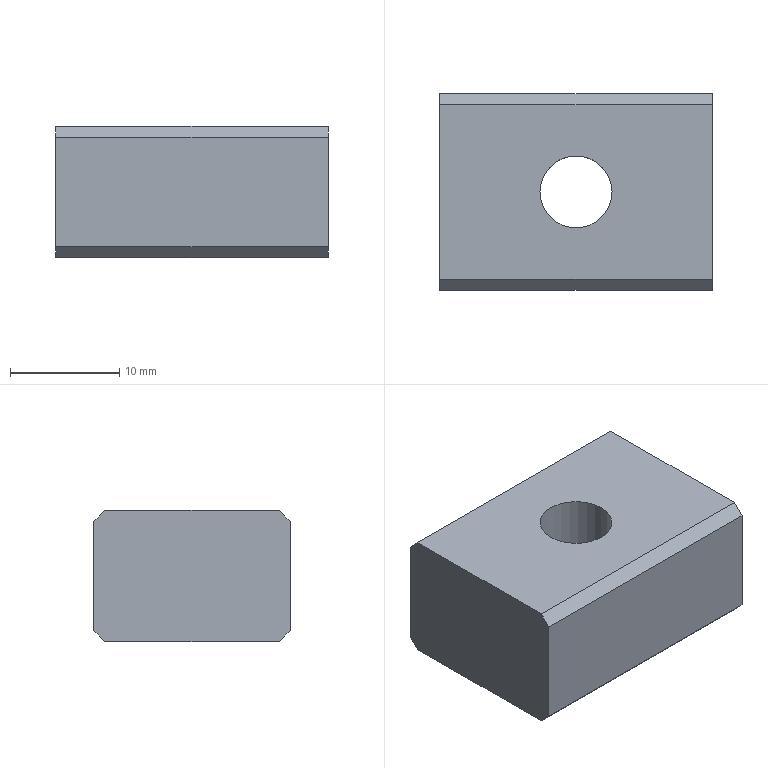Component | NX | LOCATING_KEY | 1 solid | 13 faces | box 25 x 18 x 12 mm | volume 4526 mm3 | plane 11 | cylinder 2 | commonest cylinder face diameters 6.6 x1 11 x1
STEP:
#1=CARTESIAN_POINT('',(0.,0.,0.));
#2=DIRECTION('',(0.,0.,1.));
#3=DIRECTION('',(1.,0.,0.));
#4=AXIS2_PLACEMENT_3D('',#1,#2,#3);
#5=CARTESIAN_POINT('',(195.,99.,29.));
#6=VERTEX_POINT('',#5);
#7=CARTESIAN_POINT('',(195.,99.,19.));
#8=VERTEX_POINT('',#7);
#9=CARTESIAN_POINT('',(195.,99.,30.));
#10=DIRECTION('',(0.,0.,-1.));
#11=VECTOR('',#10,1.);
#12=LINE('',#9,#11);
#13=CARTESIAN_POINT('',(195.,99.,30.));
#14=DIRECTION('',(1.,0.,0.));
#15=DIRECTION('',(0.,0.,-1.));
#16=AXIS2_PLACEMENT_3D('',#13,#14,#15);
#17=PLANE('',#16);
#18=CARTESIAN_POINT('',(0.,0.));
#19=DIRECTION('',(1.,0.));
#20=VECTOR('',#19,1.);
#21=LINE('',#18,#20);
#22=(GEOMETRIC_REPRESENTATION_CONTEXT(2)PARAMETRIC_REPRESENTATION_CONTEXT()REPRESENTATION_CONTEXT('',''));
#23=DEFINITIONAL_REPRESENTATION('',(#21),#22);
#24=PCURVE('',#17,#23);
#25=CARTESIAN_POINT('',(220.,99.,30.));
#26=DIRECTION('',(0.,-1.,0.));
#27=DIRECTION('',(0.,0.,-1.));
#28=AXIS2_PLACEMENT_3D('',#25,#26,#27);
#29=PLANE('',#28);
#30=CARTESIAN_POINT('',(0.,-25.));
#31=DIRECTION('',(1.,0.));
#32=VECTOR('',#31,1.);
#33=LINE('',#30,#32);
#34=(GEOMETRIC_REPRESENTATION_CONTEXT(2)PARAMETRIC_REPRESENTATION_CONTEXT()REPRESENTATION_CONTEXT('',''));
#35=DEFINITIONAL_REPRESENTATION('',(#33),#34);
#36=PCURVE('',#29,#35);
#37=SURFACE_CURVE('',#12,(#24,#36),.PCURVE_S1.);
#38=EDGE_CURVE('',#6,#8,#37,.T.);
#39=ORIENTED_EDGE('',*,*,#38,.T.);
#40=CARTESIAN_POINT('',(195.,98.,18.));
#41=VERTEX_POINT('',#40);
#42=CARTESIAN_POINT('',(195.,99.,19.));
#43=DIRECTION('',(0.,-0.7071,-0.7071));
#44=VECTOR('',#43,1.);
#45=LINE('',#42,#44);
#46=CARTESIAN_POINT('',(11.,0.));
#47=DIRECTION('',(0.7071,-0.7071));
#48=VECTOR('',#47,1.);
#49=LINE('',#46,#48);
#50=(GEOMETRIC_REPRESENTATION_CONTEXT(2)PARAMETRIC_REPRESENTATION_CONTEXT()REPRESENTATION_CONTEXT('',''));
#51=DEFINITIONAL_REPRESENTATION('',(#49),#50);
#52=PCURVE('',#17,#51);
#53=CARTESIAN_POINT('',(220.,99.,19.));
#54=DIRECTION('',(0.,-0.7071,0.7071));
#55=DIRECTION('',(-1.,0.,0.));
#56=AXIS2_PLACEMENT_3D('',#53,#54,#55);
#57=PLANE('',#56);
#58=CARTESIAN_POINT('',(25.,0.));
#59=DIRECTION('',(0.,1.));
#60=VECTOR('',#59,1.);
#61=LINE('',#58,#60);
#62=(GEOMETRIC_REPRESENTATION_CONTEXT(2)PARAMETRIC_REPRESENTATION_CONTEXT()REPRESENTATION_CONTEXT('',''));
#63=DEFINITIONAL_REPRESENTATION('',(#61),#62);
#64=PCURVE('',#57,#63);
#65=SURFACE_CURVE('',#45,(#52,#64),.PCURVE_S1.);
#66=EDGE_CURVE('',#8,#41,#65,.T.);
#67=ORIENTED_EDGE('',*,*,#66,.T.);
#68=CARTESIAN_POINT('',(195.,82.,18.));
#69=VERTEX_POINT('',#68);
#70=CARTESIAN_POINT('',(195.,99.,18.));
#71=DIRECTION('',(0.,-1.,0.));
#72=VECTOR('',#71,1.);
#73=LINE('',#70,#72);
#74=CARTESIAN_POINT('',(12.,0.));
#75=DIRECTION('',(0.,-1.));
#76=VECTOR('',#75,1.);
#77=LINE('',#74,#76);
#78=(GEOMETRIC_REPRESENTATION_CONTEXT(2)PARAMETRIC_REPRESENTATION_CONTEXT()REPRESENTATION_CONTEXT('',''));
#79=DEFINITIONAL_REPRESENTATION('',(#77),#78);
#80=PCURVE('',#17,#79);
#81=CARTESIAN_POINT('',(207.5,90.,18.));
#82=DIRECTION('',(0.,0.,1.));
#83=DIRECTION('',(1.,0.,0.));
#84=AXIS2_PLACEMENT_3D('',#81,#82,#83);
#85=PLANE('',#84);
#86=CARTESIAN_POINT('',(-12.5,9.));
#87=DIRECTION('',(0.,-1.));
#88=VECTOR('',#87,1.);
#89=LINE('',#86,#88);
#90=(GEOMETRIC_REPRESENTATION_CONTEXT(2)PARAMETRIC_REPRESENTATION_CONTEXT()REPRESENTATION_CONTEXT('',''));
#91=DEFINITIONAL_REPRESENTATION('',(#89),#90);
#92=PCURVE('',#85,#91);
#93=SURFACE_CURVE('',#73,(#80,#92),.PCURVE_S1.);
#94=EDGE_CURVE('',#41,#69,#93,.T.);
#95=ORIENTED_EDGE('',*,*,#94,.T.);
#96=CARTESIAN_POINT('',(195.,81.,19.));
#97=VERTEX_POINT('',#96);
#98=CARTESIAN_POINT('',(195.,81.,19.));
#99=DIRECTION('',(0.,-0.7071,0.7071));
#100=VECTOR('',#99,1.);
#101=LINE('',#98,#100);
#102=CARTESIAN_POINT('',(11.,-18.));
#103=DIRECTION('',(-0.7071,-0.7071));
#104=VECTOR('',#103,1.);
#105=LINE('',#102,#104);
#106=(GEOMETRIC_REPRESENTATION_CONTEXT(2)PARAMETRIC_REPRESENTATION_CONTEXT()REPRESENTATION_CONTEXT('',''));
#107=DEFINITIONAL_REPRESENTATION('',(#105),#106);
#108=PCURVE('',#17,#107);
#109=CARTESIAN_POINT('',(195.,81.,19.));
#110=DIRECTION('',(0.,0.7071,0.7071));
#111=DIRECTION('',(1.,0.,0.));
#112=AXIS2_PLACEMENT_3D('',#109,#110,#111);
#113=PLANE('',#112);
#114=CARTESIAN_POINT('',(0.,0.));
#115=DIRECTION('',(0.,-1.));
#116=VECTOR('',#115,1.);
#117=LINE('',#114,#116);
#118=(GEOMETRIC_REPRESENTATION_CONTEXT(2)PARAMETRIC_REPRESENTATION_CONTEXT()REPRESENTATION_CONTEXT('',''));
#119=DEFINITIONAL_REPRESENTATION('',(#117),#118);
#120=PCURVE('',#113,#119);
#121=SURFACE_CURVE('',#101,(#108,#120),.PCURVE_S1.);
#122=EDGE_CURVE('',#69,#97,#121,.T.);
#123=ORIENTED_EDGE('',*,*,#122,.T.);
#124=CARTESIAN_POINT('',(195.,81.,29.));
#125=VERTEX_POINT('',#124);
#126=CARTESIAN_POINT('',(195.,81.,30.));
#127=DIRECTION('',(0.,0.,-1.));
#128=VECTOR('',#127,1.);
#129=LINE('',#126,#128);
#130=CARTESIAN_POINT('',(0.,-18.));
#131=DIRECTION('',(1.,0.));
#132=VECTOR('',#131,1.);
#133=LINE('',#130,#132);
#134=(GEOMETRIC_REPRESENTATION_CONTEXT(2)PARAMETRIC_REPRESENTATION_CONTEXT()REPRESENTATION_CONTEXT('',''));
#135=DEFINITIONAL_REPRESENTATION('',(#133),#134);
#136=PCURVE('',#17,#135);
#137=CARTESIAN_POINT('',(195.,81.,30.));
#138=DIRECTION('',(0.,1.,0.));
#139=DIRECTION('',(0.,0.,1.));
#140=AXIS2_PLACEMENT_3D('',#137,#138,#139);
#141=PLANE('',#140);
#142=CARTESIAN_POINT('',(0.,0.));
#143=DIRECTION('',(-1.,0.));
#144=VECTOR('',#143,1.);
#145=LINE('',#142,#144);
#146=(GEOMETRIC_REPRESENTATION_CONTEXT(2)PARAMETRIC_REPRESENTATION_CONTEXT()REPRESENTATION_CONTEXT('',''));
#147=DEFINITIONAL_REPRESENTATION('',(#145),#146);
#148=PCURVE('',#141,#147);
#149=SURFACE_CURVE('',#129,(#136,#148),.PCURVE_S1.);
#150=EDGE_CURVE('',#125,#97,#149,.T.);
#151=ORIENTED_EDGE('',*,*,#150,.F.);
#152=CARTESIAN_POINT('',(195.,82.,30.));
#153=VERTEX_POINT('',#152);
#154=CARTESIAN_POINT('',(195.,82.,30.));
#155=DIRECTION('',(0.,0.7071,0.7071));
#156=VECTOR('',#155,1.);
#157=LINE('',#154,#156);
#158=CARTESIAN_POINT('',(0.,-17.));
#159=DIRECTION('',(-0.7071,0.7071));
#160=VECTOR('',#159,1.);
#161=LINE('',#158,#160);
#162=(GEOMETRIC_REPRESENTATION_CONTEXT(2)PARAMETRIC_REPRESENTATION_CONTEXT()REPRESENTATION_CONTEXT('',''));
#163=DEFINITIONAL_REPRESENTATION('',(#161),#162);
#164=PCURVE('',#17,#163);
#165=CARTESIAN_POINT('',(207.5,82.,30.));
#166=DIRECTION('',(0.,-0.7071,0.7071));
#167=DIRECTION('',(-1.,0.,0.));
#168=AXIS2_PLACEMENT_3D('',#165,#166,#167);
#169=PLANE('',#168);
#170=CARTESIAN_POINT('',(12.5,0.));
#171=DIRECTION('',(0.,-1.));
#172=VECTOR('',#171,1.);
#173=LINE('',#170,#172);
#174=(GEOMETRIC_REPRESENTATION_CONTEXT(2)PARAMETRIC_REPRESENTATION_CONTEXT()REPRESENTATION_CONTEXT('',''));
#175=DEFINITIONAL_REPRESENTATION('',(#173),#174);
#176=PCURVE('',#169,#175);
#177=SURFACE_CURVE('',#157,(#164,#176),.PCURVE_S1.);
#178=EDGE_CURVE('',#125,#153,#177,.T.);
#179=ORIENTED_EDGE('',*,*,#178,.T.);
#180=CARTESIAN_POINT('',(195.,98.,30.));
#181=VERTEX_POINT('',#180);
#182=CARTESIAN_POINT('',(195.,99.,30.));
#183=DIRECTION('',(0.,-1.,0.));
#184=VECTOR('',#183,1.);
#185=LINE('',#182,#184);
#186=CARTESIAN_POINT('',(0.,0.));
#187=DIRECTION('',(0.,-1.));
#188=VECTOR('',#187,1.);
#189=LINE('',#186,#188);
#190=(GEOMETRIC_REPRESENTATION_CONTEXT(2)PARAMETRIC_REPRESENTATION_CONTEXT()REPRESENTATION_CONTEXT('',''));
#191=DEFINITIONAL_REPRESENTATION('',(#189),#190);
#192=PCURVE('',#17,#191);
#193=CARTESIAN_POINT('',(207.5,90.,30.));
#194=DIRECTION('',(0.,0.,1.));
#195=DIRECTION('',(1.,0.,0.));
#196=AXIS2_PLACEMENT_3D('',#193,#194,#195);
#197=PLANE('',#196);
#198=CARTESIAN_POINT('',(-12.5,9.));
#199=DIRECTION('',(0.,-1.));
#200=VECTOR('',#199,1.);
#201=LINE('',#198,#200);
#202=(GEOMETRIC_REPRESENTATION_CONTEXT(2)PARAMETRIC_REPRESENTATION_CONTEXT()REPRESENTATION_CONTEXT('',''));
#203=DEFINITIONAL_REPRESENTATION('',(#201),#202);
#204=PCURVE('',#197,#203);
#205=SURFACE_CURVE('',#185,(#192,#204),.PCURVE_S1.);
#206=EDGE_CURVE('',#181,#153,#205,.T.);
#207=ORIENTED_EDGE('',*,*,#206,.F.);
#208=CARTESIAN_POINT('',(195.,98.,30.));
#209=DIRECTION('',(0.,0.7071,-0.7071));
#210=VECTOR('',#209,1.);
#211=LINE('',#208,#210);
#212=CARTESIAN_POINT('',(0.,-1.));
#213=DIRECTION('',(0.7071,0.7071));
#214=VECTOR('',#213,1.);
#215=LINE('',#212,#214);
#216=(GEOMETRIC_REPRESENTATION_CONTEXT(2)PARAMETRIC_REPRESENTATION_CONTEXT()REPRESENTATION_CONTEXT('',''));
#217=DEFINITIONAL_REPRESENTATION('',(#215),#216);
#218=PCURVE('',#17,#217);
#219=CARTESIAN_POINT('',(207.5,98.,30.));
#220=DIRECTION('',(0.,0.7071,0.7071));
#221=DIRECTION('',(1.,0.,0.));
#222=AXIS2_PLACEMENT_3D('',#219,#220,#221);
#223=PLANE('',#222);
#224=CARTESIAN_POINT('',(-12.5,0.));
#225=DIRECTION('',(0.,1.));
#226=VECTOR('',#225,1.);
#227=LINE('',#224,#226);
#228=(GEOMETRIC_REPRESENTATION_CONTEXT(2)PARAMETRIC_REPRESENTATION_CONTEXT()REPRESENTATION_CONTEXT('',''));
#229=DEFINITIONAL_REPRESENTATION('',(#227),#228);
#230=PCURVE('',#223,#229);
#231=SURFACE_CURVE('',#211,(#218,#230),.PCURVE_S1.);
#232=EDGE_CURVE('',#181,#6,#231,.T.);
#233=ORIENTED_EDGE('',*,*,#232,.T.);
#234=EDGE_LOOP('',(#39,#67,#95,#123,#151,#179,#207,#233));
#235=FACE_BOUND('',#234,.T.);
#236=ADVANCED_FACE('',(#235),#17,.F.);
#237=ORIENTED_EDGE('',*,*,#150,.T.);
#238=CARTESIAN_POINT('',(220.,81.,19.));
#239=VERTEX_POINT('',#238);
#240=CARTESIAN_POINT('',(195.,81.,19.));
#241=DIRECTION('',(1.,0.,0.));
#242=VECTOR('',#241,1.);
#243=LINE('',#240,#242);
#244=CARTESIAN_POINT('',(-11.,0.));
#245=DIRECTION('',(0.,1.));
#246=VECTOR('',#245,1.);
#247=LINE('',#244,#246);
#248=(GEOMETRIC_REPRESENTATION_CONTEXT(2)PARAMETRIC_REPRESENTATION_CONTEXT()REPRESENTATION_CONTEXT('',''));
#249=DEFINITIONAL_REPRESENTATION('',(#247),#248);
#250=PCURVE('',#141,#249);
#251=CARTESIAN_POINT('',(0.,0.));
#252=DIRECTION('',(1.,0.));
#253=VECTOR('',#252,1.);
#254=LINE('',#251,#253);
#255=(GEOMETRIC_REPRESENTATION_CONTEXT(2)PARAMETRIC_REPRESENTATION_CONTEXT()REPRESENTATION_CONTEXT('',''));
#256=DEFINITIONAL_REPRESENTATION('',(#254),#255);
#257=PCURVE('',#113,#256);
#258=SURFACE_CURVE('',#243,(#250,#257),.PCURVE_S1.);
#259=EDGE_CURVE('',#97,#239,#258,.T.);
#260=ORIENTED_EDGE('',*,*,#259,.T.);
#261=CARTESIAN_POINT('',(220.,81.,29.));
#262=VERTEX_POINT('',#261);
#263=CARTESIAN_POINT('',(220.,81.,30.));
#264=DIRECTION('',(0.,0.,-1.));
#265=VECTOR('',#264,1.);
#266=LINE('',#263,#265);
#267=CARTESIAN_POINT('',(0.,25.));
#268=DIRECTION('',(-1.,0.));
#269=VECTOR('',#268,1.);
#270=LINE('',#267,#269);
#271=(GEOMETRIC_REPRESENTATION_CONTEXT(2)PARAMETRIC_REPRESENTATION_CONTEXT()REPRESENTATION_CONTEXT('',''));
#272=DEFINITIONAL_REPRESENTATION('',(#270),#271);
#273=PCURVE('',#141,#272);
#274=CARTESIAN_POINT('',(220.,81.,30.));
#275=DIRECTION('',(-1.,0.,0.));
#276=DIRECTION('',(0.,0.,1.));
#277=AXIS2_PLACEMENT_3D('',#274,#275,#276);
#278=PLANE('',#277);
#279=CARTESIAN_POINT('',(0.,0.));
#280=DIRECTION('',(-1.,0.));
#281=VECTOR('',#280,1.);
#282=LINE('',#279,#281);
#283=(GEOMETRIC_REPRESENTATION_CONTEXT(2)PARAMETRIC_REPRESENTATION_CONTEXT()REPRESENTATION_CONTEXT('',''));
#284=DEFINITIONAL_REPRESENTATION('',(#282),#283);
#285=PCURVE('',#278,#284);
#286=SURFACE_CURVE('',#266,(#273,#285),.PCURVE_S1.);
#287=EDGE_CURVE('',#262,#239,#286,.T.);
#288=ORIENTED_EDGE('',*,*,#287,.F.);
#289=CARTESIAN_POINT('',(195.,81.,29.));
#290=DIRECTION('',(-1.,0.,0.));
#291=VECTOR('',#290,1.);
#292=LINE('',#289,#291);
#293=CARTESIAN_POINT('',(-1.,0.));
#294=DIRECTION('',(0.,-1.));
#295=VECTOR('',#294,1.);
#296=LINE('',#293,#295);
#297=(GEOMETRIC_REPRESENTATION_CONTEXT(2)PARAMETRIC_REPRESENTATION_CONTEXT()REPRESENTATION_CONTEXT('',''));
#298=DEFINITIONAL_REPRESENTATION('',(#296),#297);
#299=PCURVE('',#141,#298);
#300=CARTESIAN_POINT('',(12.5,1.414));
#301=DIRECTION('',(1.,0.));
#302=VECTOR('',#301,1.);
#303=LINE('',#300,#302);
#304=(GEOMETRIC_REPRESENTATION_CONTEXT(2)PARAMETRIC_REPRESENTATION_CONTEXT()REPRESENTATION_CONTEXT('',''));
#305=DEFINITIONAL_REPRESENTATION('',(#303),#304);
#306=PCURVE('',#169,#305);
#307=SURFACE_CURVE('',#292,(#299,#306),.PCURVE_S1.);
#308=EDGE_CURVE('',#262,#125,#307,.T.);
#309=ORIENTED_EDGE('',*,*,#308,.T.);
#310=EDGE_LOOP('',(#237,#260,#288,#309));
#311=FACE_BOUND('',#310,.T.);
#312=ADVANCED_FACE('',(#311),#141,.F.);
#313=CARTESIAN_POINT('',(220.,82.,18.));
#314=VERTEX_POINT('',#313);
#315=CARTESIAN_POINT('',(220.,98.,18.));
#316=VERTEX_POINT('',#315);
#317=CARTESIAN_POINT('',(220.,81.,18.));
#318=DIRECTION('',(0.,1.,0.));
#319=VECTOR('',#318,1.);
#320=LINE('',#317,#319);
#321=CARTESIAN_POINT('',(-12.,0.));
#322=DIRECTION('',(0.,1.));
#323=VECTOR('',#322,1.);
#324=LINE('',#321,#323);
#325=(GEOMETRIC_REPRESENTATION_CONTEXT(2)PARAMETRIC_REPRESENTATION_CONTEXT()REPRESENTATION_CONTEXT('',''));
#326=DEFINITIONAL_REPRESENTATION('',(#324),#325);
#327=PCURVE('',#278,#326);
#328=CARTESIAN_POINT('',(12.5,-9.));
#329=DIRECTION('',(0.,1.));
#330=VECTOR('',#329,1.);
#331=LINE('',#328,#330);
#332=(GEOMETRIC_REPRESENTATION_CONTEXT(2)PARAMETRIC_REPRESENTATION_CONTEXT()REPRESENTATION_CONTEXT('',''));
#333=DEFINITIONAL_REPRESENTATION('',(#331),#332);
#334=PCURVE('',#85,#333);
#335=SURFACE_CURVE('',#320,(#327,#334),.PCURVE_S1.);
#336=EDGE_CURVE('',#314,#316,#335,.T.);
#337=ORIENTED_EDGE('',*,*,#336,.T.);
#338=CARTESIAN_POINT('',(220.,99.,19.));
#339=VERTEX_POINT('',#338);
#340=CARTESIAN_POINT('',(220.,99.,19.));
#341=DIRECTION('',(0.,0.7071,0.7071));
#342=VECTOR('',#341,1.);
#343=LINE('',#340,#342);
#344=CARTESIAN_POINT('',(-11.,18.));
#345=DIRECTION('',(0.7071,0.7071));
#346=VECTOR('',#345,1.);
#347=LINE('',#344,#346);
#348=(GEOMETRIC_REPRESENTATION_CONTEXT(2)PARAMETRIC_REPRESENTATION_CONTEXT()REPRESENTATION_CONTEXT('',''));
#349=DEFINITIONAL_REPRESENTATION('',(#347),#348);
#350=PCURVE('',#278,#349);
#351=CARTESIAN_POINT('',(0.,0.));
#352=DIRECTION('',(0.,-1.));
#353=VECTOR('',#352,1.);
#354=LINE('',#351,#353);
#355=(GEOMETRIC_REPRESENTATION_CONTEXT(2)PARAMETRIC_REPRESENTATION_CONTEXT()REPRESENTATION_CONTEXT('',''));
#356=DEFINITIONAL_REPRESENTATION('',(#354),#355);
#357=PCURVE('',#57,#356);
#358=SURFACE_CURVE('',#343,(#350,#357),.PCURVE_S1.);
#359=EDGE_CURVE('',#316,#339,#358,.T.);
#360=ORIENTED_EDGE('',*,*,#359,.T.);
#361=CARTESIAN_POINT('',(220.,99.,29.));
#362=VERTEX_POINT('',#361);
#363=CARTESIAN_POINT('',(220.,99.,30.));
#364=DIRECTION('',(0.,0.,-1.));
#365=VECTOR('',#364,1.);
#366=LINE('',#363,#365);
#367=CARTESIAN_POINT('',(0.,18.));
#368=DIRECTION('',(-1.,0.));
#369=VECTOR('',#368,1.);
#370=LINE('',#367,#369);
#371=(GEOMETRIC_REPRESENTATION_CONTEXT(2)PARAMETRIC_REPRESENTATION_CONTEXT()REPRESENTATION_CONTEXT('',''));
#372=DEFINITIONAL_REPRESENTATION('',(#370),#371);
#373=PCURVE('',#278,#372);
#374=CARTESIAN_POINT('',(0.,0.));
#375=DIRECTION('',(1.,0.));
#376=VECTOR('',#375,1.);
#377=LINE('',#374,#376);
#378=(GEOMETRIC_REPRESENTATION_CONTEXT(2)PARAMETRIC_REPRESENTATION_CONTEXT()REPRESENTATION_CONTEXT('',''));
#379=DEFINITIONAL_REPRESENTATION('',(#377),#378);
#380=PCURVE('',#29,#379);
#381=SURFACE_CURVE('',#366,(#373,#380),.PCURVE_S1.);
#382=EDGE_CURVE('',#362,#339,#381,.T.);
#383=ORIENTED_EDGE('',*,*,#382,.F.);
#384=CARTESIAN_POINT('',(220.,98.,30.));
#385=VERTEX_POINT('',#384);
#386=CARTESIAN_POINT('',(220.,98.,30.));
#387=DIRECTION('',(0.,-0.7071,0.7071));
#388=VECTOR('',#387,1.);
#389=LINE('',#386,#388);
#390=CARTESIAN_POINT('',(0.,17.));
#391=DIRECTION('',(0.7071,-0.7071));
#392=VECTOR('',#391,1.);
#393=LINE('',#390,#392);
#394=(GEOMETRIC_REPRESENTATION_CONTEXT(2)PARAMETRIC_REPRESENTATION_CONTEXT()REPRESENTATION_CONTEXT('',''));
#395=DEFINITIONAL_REPRESENTATION('',(#393),#394);
#396=PCURVE('',#278,#395);
#397=CARTESIAN_POINT('',(12.5,0.));
#398=DIRECTION('',(0.,-1.));
#399=VECTOR('',#398,1.);
#400=LINE('',#397,#399);
#401=(GEOMETRIC_REPRESENTATION_CONTEXT(2)PARAMETRIC_REPRESENTATION_CONTEXT()REPRESENTATION_CONTEXT('',''));
#402=DEFINITIONAL_REPRESENTATION('',(#400),#401);
#403=PCURVE('',#223,#402);
#404=SURFACE_CURVE('',#389,(#396,#403),.PCURVE_S1.);
#405=EDGE_CURVE('',#362,#385,#404,.T.);
#406=ORIENTED_EDGE('',*,*,#405,.T.);
#407=CARTESIAN_POINT('',(220.,82.,30.));
#408=VERTEX_POINT('',#407);
#409=CARTESIAN_POINT('',(220.,81.,30.));
#410=DIRECTION('',(0.,1.,0.));
#411=VECTOR('',#410,1.);
#412=LINE('',#409,#411);
#413=CARTESIAN_POINT('',(0.,0.));
#414=DIRECTION('',(0.,1.));
#415=VECTOR('',#414,1.);
#416=LINE('',#413,#415);
#417=(GEOMETRIC_REPRESENTATION_CONTEXT(2)PARAMETRIC_REPRESENTATION_CONTEXT()REPRESENTATION_CONTEXT('',''));
#418=DEFINITIONAL_REPRESENTATION('',(#416),#417);
#419=PCURVE('',#278,#418);
#420=CARTESIAN_POINT('',(12.5,-9.));
#421=DIRECTION('',(0.,1.));
#422=VECTOR('',#421,1.);
#423=LINE('',#420,#422);
#424=(GEOMETRIC_REPRESENTATION_CONTEXT(2)PARAMETRIC_REPRESENTATION_CONTEXT()REPRESENTATION_CONTEXT('',''));
#425=DEFINITIONAL_REPRESENTATION('',(#423),#424);
#426=PCURVE('',#197,#425);
#427=SURFACE_CURVE('',#412,(#419,#426),.PCURVE_S1.);
#428=EDGE_CURVE('',#408,#385,#427,.T.);
#429=ORIENTED_EDGE('',*,*,#428,.F.);
#430=CARTESIAN_POINT('',(220.,82.,30.));
#431=DIRECTION('',(0.,-0.7071,-0.7071));
#432=VECTOR('',#431,1.);
#433=LINE('',#430,#432);
#434=CARTESIAN_POINT('',(0.,1.));
#435=DIRECTION('',(-0.7071,-0.7071));
#436=VECTOR('',#435,1.);
#437=LINE('',#434,#436);
#438=(GEOMETRIC_REPRESENTATION_CONTEXT(2)PARAMETRIC_REPRESENTATION_CONTEXT()REPRESENTATION_CONTEXT('',''));
#439=DEFINITIONAL_REPRESENTATION('',(#437),#438);
#440=PCURVE('',#278,#439);
#441=CARTESIAN_POINT('',(-12.5,0.));
#442=DIRECTION('',(0.,1.));
#443=VECTOR('',#442,1.);
#444=LINE('',#441,#443);
#445=(GEOMETRIC_REPRESENTATION_CONTEXT(2)PARAMETRIC_REPRESENTATION_CONTEXT()REPRESENTATION_CONTEXT('',''));
#446=DEFINITIONAL_REPRESENTATION('',(#444),#445);
#447=PCURVE('',#169,#446);
#448=SURFACE_CURVE('',#433,(#440,#447),.PCURVE_S1.);
#449=EDGE_CURVE('',#408,#262,#448,.T.);
#450=ORIENTED_EDGE('',*,*,#449,.T.);
#451=ORIENTED_EDGE('',*,*,#287,.T.);
#452=CARTESIAN_POINT('',(220.,81.,19.));
#453=DIRECTION('',(0.,0.7071,-0.7071));
#454=VECTOR('',#453,1.);
#455=LINE('',#452,#454);
#456=CARTESIAN_POINT('',(-11.,0.));
#457=DIRECTION('',(-0.7071,0.7071));
#458=VECTOR('',#457,1.);
#459=LINE('',#456,#458);
#460=(GEOMETRIC_REPRESENTATION_CONTEXT(2)PARAMETRIC_REPRESENTATION_CONTEXT()REPRESENTATION_CONTEXT('',''));
#461=DEFINITIONAL_REPRESENTATION('',(#459),#460);
#462=PCURVE('',#278,#461);
#463=CARTESIAN_POINT('',(25.,0.));
#464=DIRECTION('',(0.,1.));
#465=VECTOR('',#464,1.);
#466=LINE('',#463,#465);
#467=(GEOMETRIC_REPRESENTATION_CONTEXT(2)PARAMETRIC_REPRESENTATION_CONTEXT()REPRESENTATION_CONTEXT('',''));
#468=DEFINITIONAL_REPRESENTATION('',(#466),#467);
#469=PCURVE('',#113,#468);
#470=SURFACE_CURVE('',#455,(#462,#469),.PCURVE_S1.);
#471=EDGE_CURVE('',#239,#314,#470,.T.);
#472=ORIENTED_EDGE('',*,*,#471,.T.);
#473=EDGE_LOOP('',(#337,#360,#383,#406,#429,#450,#451,#472));
#474=FACE_BOUND('',#473,.T.);
#475=ADVANCED_FACE('',(#474),#278,.F.);
#476=ORIENTED_EDGE('',*,*,#382,.T.);
#477=CARTESIAN_POINT('',(220.,99.,19.));
#478=DIRECTION('',(-1.,0.,0.));
#479=VECTOR('',#478,1.);
#480=LINE('',#477,#479);
#481=CARTESIAN_POINT('',(11.,0.));
#482=DIRECTION('',(0.,-1.));
#483=VECTOR('',#482,1.);
#484=LINE('',#481,#483);
#485=(GEOMETRIC_REPRESENTATION_CONTEXT(2)PARAMETRIC_REPRESENTATION_CONTEXT()REPRESENTATION_CONTEXT('',''));
#486=DEFINITIONAL_REPRESENTATION('',(#484),#485);
#487=PCURVE('',#29,#486);
#488=CARTESIAN_POINT('',(0.,0.));
#489=DIRECTION('',(1.,0.));
#490=VECTOR('',#489,1.);
#491=LINE('',#488,#490);
#492=(GEOMETRIC_REPRESENTATION_CONTEXT(2)PARAMETRIC_REPRESENTATION_CONTEXT()REPRESENTATION_CONTEXT('',''));
#493=DEFINITIONAL_REPRESENTATION('',(#491),#492);
#494=PCURVE('',#57,#493);
#495=SURFACE_CURVE('',#480,(#487,#494),.PCURVE_S1.);
#496=EDGE_CURVE('',#339,#8,#495,.T.);
#497=ORIENTED_EDGE('',*,*,#496,.T.);
#498=ORIENTED_EDGE('',*,*,#38,.F.);
#499=CARTESIAN_POINT('',(220.,99.,29.));
#500=DIRECTION('',(1.,0.,0.));
#501=VECTOR('',#500,1.);
#502=LINE('',#499,#501);
#503=CARTESIAN_POINT('',(1.,0.));
#504=DIRECTION('',(0.,1.));
#505=VECTOR('',#504,1.);
#506=LINE('',#503,#505);
#507=(GEOMETRIC_REPRESENTATION_CONTEXT(2)PARAMETRIC_REPRESENTATION_CONTEXT()REPRESENTATION_CONTEXT('',''));
#508=DEFINITIONAL_REPRESENTATION('',(#506),#507);
#509=PCURVE('',#29,#508);
#510=CARTESIAN_POINT('',(12.5,1.414));
#511=DIRECTION('',(1.,0.));
#512=VECTOR('',#511,1.);
#513=LINE('',#510,#512);
#514=(GEOMETRIC_REPRESENTATION_CONTEXT(2)PARAMETRIC_REPRESENTATION_CONTEXT()REPRESENTATION_CONTEXT('',''));
#515=DEFINITIONAL_REPRESENTATION('',(#513),#514);
#516=PCURVE('',#223,#515);
#517=SURFACE_CURVE('',#502,(#509,#516),.PCURVE_S1.);
#518=EDGE_CURVE('',#6,#362,#517,.T.);
#519=ORIENTED_EDGE('',*,*,#518,.T.);
#520=EDGE_LOOP('',(#476,#497,#498,#519));
#521=FACE_BOUND('',#520,.T.);
#522=ADVANCED_FACE('',(#521),#29,.F.);
#523=CARTESIAN_POINT('',(210.8,90.,30.));
#524=VERTEX_POINT('',#523);
#525=CARTESIAN_POINT('',(207.5,90.,30.));
#526=DIRECTION('',(0.,0.,1.));
#527=DIRECTION('',(1.,0.,0.));
#528=AXIS2_PLACEMENT_3D('',#525,#526,#527);
#529=CIRCLE('',#528,3.3);
#530=CARTESIAN_POINT('',(0.,0.));
#531=DIRECTION('',(1.,0.));
#532=AXIS2_PLACEMENT_2D('',#530,#531);
#533=CIRCLE('',#532,3.3);
#534=(GEOMETRIC_REPRESENTATION_CONTEXT(2)PARAMETRIC_REPRESENTATION_CONTEXT()REPRESENTATION_CONTEXT('',''));
#535=DEFINITIONAL_REPRESENTATION('',(#533),#534);
#536=PCURVE('',#197,#535);
#537=CARTESIAN_POINT('',(207.5,90.,42.183));
#538=DIRECTION('',(0.,0.,1.));
#539=DIRECTION('',(1.,0.,0.));
#540=AXIS2_PLACEMENT_3D('',#537,#538,#539);
#541=CYLINDRICAL_SURFACE('',#540,3.3);
#542=CARTESIAN_POINT('',(0.,-12.183));
#543=DIRECTION('',(1.,0.));
#544=VECTOR('',#543,1.);
#545=LINE('',#542,#544);
#546=(GEOMETRIC_REPRESENTATION_CONTEXT(2)PARAMETRIC_REPRESENTATION_CONTEXT()REPRESENTATION_CONTEXT('',''));
#547=DEFINITIONAL_REPRESENTATION('',(#545),#546);
#548=PCURVE('',#541,#547);
#549=SURFACE_CURVE('',#529,(#536,#548),.PCURVE_S1.);
#550=EDGE_CURVE('',#524,#524,#549,.T.);
#551=ORIENTED_EDGE('',*,*,#550,.F.);
#552=EDGE_LOOP('',(#551));
#553=FACE_BOUND('',#552,.T.);
#554=ORIENTED_EDGE('',*,*,#428,.T.);
#555=CARTESIAN_POINT('',(195.,98.,30.));
#556=DIRECTION('',(-1.,0.,0.));
#557=VECTOR('',#556,1.);
#558=LINE('',#555,#557);
#559=CARTESIAN_POINT('',(-12.5,8.));
#560=DIRECTION('',(-1.,0.));
#561=VECTOR('',#560,1.);
#562=LINE('',#559,#561);
#563=(GEOMETRIC_REPRESENTATION_CONTEXT(2)PARAMETRIC_REPRESENTATION_CONTEXT()REPRESENTATION_CONTEXT('',''));
#564=DEFINITIONAL_REPRESENTATION('',(#562),#563);
#565=PCURVE('',#197,#564);
#566=CARTESIAN_POINT('',(-12.5,0.));
#567=DIRECTION('',(-1.,0.));
#568=VECTOR('',#567,1.);
#569=LINE('',#566,#568);
#570=(GEOMETRIC_REPRESENTATION_CONTEXT(2)PARAMETRIC_REPRESENTATION_CONTEXT()REPRESENTATION_CONTEXT('',''));
#571=DEFINITIONAL_REPRESENTATION('',(#569),#570);
#572=PCURVE('',#223,#571);
#573=SURFACE_CURVE('',#558,(#565,#572),.PCURVE_S1.);
#574=EDGE_CURVE('',#385,#181,#573,.T.);
#575=ORIENTED_EDGE('',*,*,#574,.T.);
#576=ORIENTED_EDGE('',*,*,#206,.T.);
#577=CARTESIAN_POINT('',(220.,82.,30.));
#578=DIRECTION('',(1.,0.,0.));
#579=VECTOR('',#578,1.);
#580=LINE('',#577,#579);
#581=CARTESIAN_POINT('',(12.5,-8.));
#582=DIRECTION('',(1.,0.));
#583=VECTOR('',#582,1.);
#584=LINE('',#581,#583);
#585=(GEOMETRIC_REPRESENTATION_CONTEXT(2)PARAMETRIC_REPRESENTATION_CONTEXT()REPRESENTATION_CONTEXT('',''));
#586=DEFINITIONAL_REPRESENTATION('',(#584),#585);
#587=PCURVE('',#197,#586);
#588=CARTESIAN_POINT('',(-12.5,0.));
#589=DIRECTION('',(-1.,0.));
#590=VECTOR('',#589,1.);
#591=LINE('',#588,#590);
#592=(GEOMETRIC_REPRESENTATION_CONTEXT(2)PARAMETRIC_REPRESENTATION_CONTEXT()REPRESENTATION_CONTEXT('',''));
#593=DEFINITIONAL_REPRESENTATION('',(#591),#592);
#594=PCURVE('',#169,#593);
#595=SURFACE_CURVE('',#580,(#587,#594),.PCURVE_S1.);
#596=EDGE_CURVE('',#153,#408,#595,.T.);
#597=ORIENTED_EDGE('',*,*,#596,.T.);
#598=EDGE_LOOP('',(#554,#575,#576,#597));
#599=FACE_BOUND('',#598,.T.);
#600=ADVANCED_FACE('',(#553,#599),#197,.T.);
#601=CARTESIAN_POINT('',(213.,90.,18.));
#602=VERTEX_POINT('',#601);
#603=CARTESIAN_POINT('',(207.5,90.,18.));
#604=DIRECTION('',(0.,0.,1.));
#605=DIRECTION('',(1.,0.,0.));
#606=AXIS2_PLACEMENT_3D('',#603,#604,#605);
#607=CIRCLE('',#606,5.5);
#608=CARTESIAN_POINT('',(0.,0.));
#609=DIRECTION('',(1.,0.));
#610=AXIS2_PLACEMENT_2D('',#608,#609);
#611=CIRCLE('',#610,5.5);
#612=(GEOMETRIC_REPRESENTATION_CONTEXT(2)PARAMETRIC_REPRESENTATION_CONTEXT()REPRESENTATION_CONTEXT('',''));
#613=DEFINITIONAL_REPRESENTATION('',(#611),#612);
#614=PCURVE('',#85,#613);
#615=CARTESIAN_POINT('',(207.5,90.,18.));
#616=DIRECTION('',(0.,0.,1.));
#617=DIRECTION('',(1.,0.,0.));
#618=AXIS2_PLACEMENT_3D('',#615,#616,#617);
#619=CYLINDRICAL_SURFACE('',#618,5.5);
#620=CARTESIAN_POINT('',(0.,0.));
#621=DIRECTION('',(1.,0.));
#622=VECTOR('',#621,1.);
#623=LINE('',#620,#622);
#624=(GEOMETRIC_REPRESENTATION_CONTEXT(2)PARAMETRIC_REPRESENTATION_CONTEXT()REPRESENTATION_CONTEXT('',''));
#625=DEFINITIONAL_REPRESENTATION('',(#623),#624);
#626=PCURVE('',#619,#625);
#627=SURFACE_CURVE('',#607,(#614,#626),.PCURVE_S1.);
#628=EDGE_CURVE('',#602,#602,#627,.T.);
#629=ORIENTED_EDGE('',*,*,#628,.T.);
#630=EDGE_LOOP('',(#629));
#631=FACE_BOUND('',#630,.T.);
#632=ORIENTED_EDGE('',*,*,#94,.F.);
#633=CARTESIAN_POINT('',(207.5,98.,18.));
#634=DIRECTION('',(1.,0.,0.));
#635=VECTOR('',#634,1.);
#636=LINE('',#633,#635);
#637=CARTESIAN_POINT('',(0.,8.));
#638=DIRECTION('',(1.,0.));
#639=VECTOR('',#638,1.);
#640=LINE('',#637,#639);
#641=(GEOMETRIC_REPRESENTATION_CONTEXT(2)PARAMETRIC_REPRESENTATION_CONTEXT()REPRESENTATION_CONTEXT('',''));
#642=DEFINITIONAL_REPRESENTATION('',(#640),#641);
#643=PCURVE('',#85,#642);
#644=CARTESIAN_POINT('',(12.5,1.414));
#645=DIRECTION('',(-1.,0.));
#646=VECTOR('',#645,1.);
#647=LINE('',#644,#646);
#648=(GEOMETRIC_REPRESENTATION_CONTEXT(2)PARAMETRIC_REPRESENTATION_CONTEXT()REPRESENTATION_CONTEXT('',''));
#649=DEFINITIONAL_REPRESENTATION('',(#647),#648);
#650=PCURVE('',#57,#649);
#651=SURFACE_CURVE('',#636,(#643,#650),.PCURVE_S1.);
#652=EDGE_CURVE('',#41,#316,#651,.T.);
#653=ORIENTED_EDGE('',*,*,#652,.T.);
#654=ORIENTED_EDGE('',*,*,#336,.F.);
#655=CARTESIAN_POINT('',(207.5,82.,18.));
#656=DIRECTION('',(-1.,0.,0.));
#657=VECTOR('',#656,1.);
#658=LINE('',#655,#657);
#659=CARTESIAN_POINT('',(0.,-8.));
#660=DIRECTION('',(-1.,0.));
#661=VECTOR('',#660,1.);
#662=LINE('',#659,#661);
#663=(GEOMETRIC_REPRESENTATION_CONTEXT(2)PARAMETRIC_REPRESENTATION_CONTEXT()REPRESENTATION_CONTEXT('',''));
#664=DEFINITIONAL_REPRESENTATION('',(#662),#663);
#665=PCURVE('',#85,#664);
#666=CARTESIAN_POINT('',(12.5,1.414));
#667=DIRECTION('',(-1.,0.));
#668=VECTOR('',#667,1.);
#669=LINE('',#666,#668);
#670=(GEOMETRIC_REPRESENTATION_CONTEXT(2)PARAMETRIC_REPRESENTATION_CONTEXT()REPRESENTATION_CONTEXT('',''));
#671=DEFINITIONAL_REPRESENTATION('',(#669),#670);
#672=PCURVE('',#113,#671);
#673=SURFACE_CURVE('',#658,(#665,#672),.PCURVE_S1.);
#674=EDGE_CURVE('',#314,#69,#673,.T.);
#675=ORIENTED_EDGE('',*,*,#674,.T.);
#676=EDGE_LOOP('',(#632,#653,#654,#675));
#677=FACE_BOUND('',#676,.T.);
#678=ADVANCED_FACE('',(#631,#677),#85,.F.);
#679=ORIENTED_EDGE('',*,*,#550,.F.);
#680=CARTESIAN_POINT('',(210.8,90.,24.8));
#681=VERTEX_POINT('',#680);
#682=CARTESIAN_POINT('',(210.8,90.,24.8));
#683=CARTESIAN_POINT('',(210.8,90.,30.));
#684=B_SPLINE_CURVE_WITH_KNOTS('',1,(#682,#683),.UNSPECIFIED.,.F.,.F.,(2,2),(-17.383,-12.183),.PIECEWISE_BEZIER_KNOTS.);
#685=CARTESIAN_POINT('',(0.,0.));
#686=DIRECTION('',(0.,1.));
#687=VECTOR('',#686,1.);
#688=LINE('',#685,#687);
#689=(GEOMETRIC_REPRESENTATION_CONTEXT(2)PARAMETRIC_REPRESENTATION_CONTEXT()REPRESENTATION_CONTEXT('',''));
#690=DEFINITIONAL_REPRESENTATION('',(#688),#689);
#691=PCURVE('',#541,#690);
#692=CARTESIAN_POINT('',(6.283,0.));
#693=DIRECTION('',(0.,1.));
#694=VECTOR('',#693,1.);
#695=LINE('',#692,#694);
#696=(GEOMETRIC_REPRESENTATION_CONTEXT(2)PARAMETRIC_REPRESENTATION_CONTEXT()REPRESENTATION_CONTEXT('',''));
#697=DEFINITIONAL_REPRESENTATION('',(#695),#696);
#698=PCURVE('',#541,#697);
#699=SEAM_CURVE('',#684,(#691,#698),.PCURVE_S1.);
#700=EDGE_CURVE('',#681,#524,#699,.T.);
#701=ORIENTED_EDGE('',*,*,#700,.F.);
#702=CARTESIAN_POINT('',(207.5,90.,24.8));
#703=DIRECTION('',(0.,0.,-1.));
#704=DIRECTION('',(1.,0.,0.));
#705=AXIS2_PLACEMENT_3D('',#702,#703,#704);
#706=CIRCLE('',#705,3.3);
#707=CARTESIAN_POINT('',(6.283,-17.383));
#708=DIRECTION('',(-1.,0.));
#709=VECTOR('',#708,1.);
#710=LINE('',#707,#709);
#711=(GEOMETRIC_REPRESENTATION_CONTEXT(2)PARAMETRIC_REPRESENTATION_CONTEXT()REPRESENTATION_CONTEXT('',''));
#712=DEFINITIONAL_REPRESENTATION('',(#710),#711);
#713=PCURVE('',#541,#712);
#714=CARTESIAN_POINT('',(207.5,90.,24.8));
#715=DIRECTION('',(0.,0.,1.));
#716=DIRECTION('',(1.,0.,0.));
#717=AXIS2_PLACEMENT_3D('',#714,#715,#716);
#718=PLANE('',#717);
#719=CARTESIAN_POINT('',(3.3,0.));
#720=CARTESIAN_POINT('',(3.3,-5.716));
#721=CARTESIAN_POINT('',(-1.65,-2.858));
#722=CARTESIAN_POINT('',(-6.6,-0.));
#723=CARTESIAN_POINT('',(-1.65,2.858));
#724=CARTESIAN_POINT('',(3.3,5.716));
#725=CARTESIAN_POINT('',(3.3,0.));
#726=(BOUNDED_CURVE()B_SPLINE_CURVE(2,(#719,#720,#721,#722,#723,#724,#725),.UNSPECIFIED.,.T.,.F.)B_SPLINE_CURVE_WITH_KNOTS((1,2,2,2,2,1),(-2.094,0.,2.094,4.189,6.283,8.378),.UNSPECIFIED.)CURVE()GEOMETRIC_REPRESENTATION_ITEM()RATIONAL_B_SPLINE_CURVE((1.,0.5,1.,0.5,1.,0.5,1.))REPRESENTATION_ITEM(''));
#727=(GEOMETRIC_REPRESENTATION_CONTEXT(2)PARAMETRIC_REPRESENTATION_CONTEXT()REPRESENTATION_CONTEXT('',''));
#728=DEFINITIONAL_REPRESENTATION('',(#726),#727);
#729=PCURVE('',#718,#728);
#730=SURFACE_CURVE('',#706,(#713,#729),.PCURVE_S1.);
#731=EDGE_CURVE('',#681,#681,#730,.T.);
#732=ORIENTED_EDGE('',*,*,#731,.F.);
#733=ORIENTED_EDGE('',*,*,#700,.T.);
#734=EDGE_LOOP('',(#679,#701,#732,#733));
#735=FACE_BOUND('',#734,.F.);
#736=ADVANCED_FACE('',(#735),#541,.F.);
#737=ORIENTED_EDGE('',*,*,#731,.F.);
#738=EDGE_LOOP('',(#737));
#739=FACE_BOUND('',#738,.T.);
#740=CARTESIAN_POINT('',(213.,90.,24.8));
#741=VERTEX_POINT('',#740);
#742=CARTESIAN_POINT('',(207.5,90.,24.8));
#743=DIRECTION('',(0.,0.,-1.));
#744=DIRECTION('',(1.,0.,0.));
#745=AXIS2_PLACEMENT_3D('',#742,#743,#744);
#746=CIRCLE('',#745,5.5);
#747=CARTESIAN_POINT('',(5.5,0.));
#748=CARTESIAN_POINT('',(5.5,-9.526));
#749=CARTESIAN_POINT('',(-2.75,-4.763));
#750=CARTESIAN_POINT('',(-11.,-0.));
#751=CARTESIAN_POINT('',(-2.75,4.763));
#752=CARTESIAN_POINT('',(5.5,9.526));
#753=CARTESIAN_POINT('',(5.5,0.));
#754=(BOUNDED_CURVE()B_SPLINE_CURVE(2,(#747,#748,#749,#750,#751,#752,#753),.UNSPECIFIED.,.T.,.F.)B_SPLINE_CURVE_WITH_KNOTS((1,2,2,2,2,1),(-2.094,0.,2.094,4.189,6.283,8.378),.UNSPECIFIED.)CURVE()GEOMETRIC_REPRESENTATION_ITEM()RATIONAL_B_SPLINE_CURVE((1.,0.5,1.,0.5,1.,0.5,1.))REPRESENTATION_ITEM(''));
#755=(GEOMETRIC_REPRESENTATION_CONTEXT(2)PARAMETRIC_REPRESENTATION_CONTEXT()REPRESENTATION_CONTEXT('',''));
#756=DEFINITIONAL_REPRESENTATION('',(#754),#755);
#757=PCURVE('',#718,#756);
#758=CARTESIAN_POINT('',(6.283,6.8));
#759=DIRECTION('',(-1.,0.));
#760=VECTOR('',#759,1.);
#761=LINE('',#758,#760);
#762=(GEOMETRIC_REPRESENTATION_CONTEXT(2)PARAMETRIC_REPRESENTATION_CONTEXT()REPRESENTATION_CONTEXT('',''));
#763=DEFINITIONAL_REPRESENTATION('',(#761),#762);
#764=PCURVE('',#619,#763);
#765=SURFACE_CURVE('',#746,(#757,#764),.PCURVE_S1.);
#766=EDGE_CURVE('',#741,#741,#765,.T.);
#767=ORIENTED_EDGE('',*,*,#766,.T.);
#768=EDGE_LOOP('',(#767));
#769=FACE_BOUND('',#768,.T.);
#770=ADVANCED_FACE('',(#739,#769),#718,.F.);
#771=ORIENTED_EDGE('',*,*,#766,.T.);
#772=CARTESIAN_POINT('',(213.,90.,18.));
#773=CARTESIAN_POINT('',(213.,90.,24.8));
#774=B_SPLINE_CURVE_WITH_KNOTS('',1,(#772,#773),.UNSPECIFIED.,.F.,.F.,(2,2),(0.,6.8),.PIECEWISE_BEZIER_KNOTS.);
#775=CARTESIAN_POINT('',(0.,0.));
#776=DIRECTION('',(0.,1.));
#777=VECTOR('',#776,1.);
#778=LINE('',#775,#777);
#779=(GEOMETRIC_REPRESENTATION_CONTEXT(2)PARAMETRIC_REPRESENTATION_CONTEXT()REPRESENTATION_CONTEXT('',''));
#780=DEFINITIONAL_REPRESENTATION('',(#778),#779);
#781=PCURVE('',#619,#780);
#782=CARTESIAN_POINT('',(6.283,0.));
#783=DIRECTION('',(0.,1.));
#784=VECTOR('',#783,1.);
#785=LINE('',#782,#784);
#786=(GEOMETRIC_REPRESENTATION_CONTEXT(2)PARAMETRIC_REPRESENTATION_CONTEXT()REPRESENTATION_CONTEXT('',''));
#787=DEFINITIONAL_REPRESENTATION('',(#785),#786);
#788=PCURVE('',#619,#787);
#789=SEAM_CURVE('',#774,(#781,#788),.PCURVE_S1.);
#790=EDGE_CURVE('',#602,#741,#789,.T.);
#791=ORIENTED_EDGE('',*,*,#790,.F.);
#792=ORIENTED_EDGE('',*,*,#628,.T.);
#793=ORIENTED_EDGE('',*,*,#790,.T.);
#794=EDGE_LOOP('',(#771,#791,#792,#793));
#795=FACE_BOUND('',#794,.F.);
#796=ADVANCED_FACE('',(#795),#619,.F.);
#797=ORIENTED_EDGE('',*,*,#359,.F.);
#798=ORIENTED_EDGE('',*,*,#652,.F.);
#799=ORIENTED_EDGE('',*,*,#66,.F.);
#800=ORIENTED_EDGE('',*,*,#496,.F.);
#801=EDGE_LOOP('',(#797,#798,#799,#800));
#802=FACE_BOUND('',#801,.T.);
#803=ADVANCED_FACE('',(#802),#57,.F.);
#804=ORIENTED_EDGE('',*,*,#405,.F.);
#805=ORIENTED_EDGE('',*,*,#518,.F.);
#806=ORIENTED_EDGE('',*,*,#232,.F.);
#807=ORIENTED_EDGE('',*,*,#574,.F.);
#808=EDGE_LOOP('',(#804,#805,#806,#807));
#809=FACE_BOUND('',#808,.T.);
#810=ADVANCED_FACE('',(#809),#223,.T.);
#811=ORIENTED_EDGE('',*,*,#122,.F.);
#812=ORIENTED_EDGE('',*,*,#674,.F.);
#813=ORIENTED_EDGE('',*,*,#471,.F.);
#814=ORIENTED_EDGE('',*,*,#259,.F.);
#815=EDGE_LOOP('',(#811,#812,#813,#814));
#816=FACE_BOUND('',#815,.T.);
#817=ADVANCED_FACE('',(#816),#113,.F.);
#818=ORIENTED_EDGE('',*,*,#178,.F.);
#819=ORIENTED_EDGE('',*,*,#308,.F.);
#820=ORIENTED_EDGE('',*,*,#449,.F.);
#821=ORIENTED_EDGE('',*,*,#596,.F.);
#822=EDGE_LOOP('',(#818,#819,#820,#821));
#823=FACE_BOUND('',#822,.T.);
#824=ADVANCED_FACE('',(#823),#169,.T.);
#825=CLOSED_SHELL('',(#236,#312,#475,#522,#600,#678,#736,#770,#796,#803,#810,#817,#824));
#826=MANIFOLD_SOLID_BREP('',#825);
#827=(LENGTH_UNIT()NAMED_UNIT(*)SI_UNIT(.MILLI.,.METRE.));
#828=UNCERTAINTY_MEASURE_WITH_UNIT(LENGTH_MEASURE(0.000002),#827,'','');
#829=(NAMED_UNIT(*)PLANE_ANGLE_UNIT()SI_UNIT($,.RADIAN.));
#830=(NAMED_UNIT(*)SI_UNIT($,.STERADIAN.)SOLID_ANGLE_UNIT());
#831=(GEOMETRIC_REPRESENTATION_CONTEXT(3)GLOBAL_UNCERTAINTY_ASSIGNED_CONTEXT((#828))GLOBAL_UNIT_ASSIGNED_CONTEXT((#827,#829,#830))REPRESENTATION_CONTEXT('',''));
#832=ADVANCED_BREP_SHAPE_REPRESENTATION('',(#4,#826),#831);